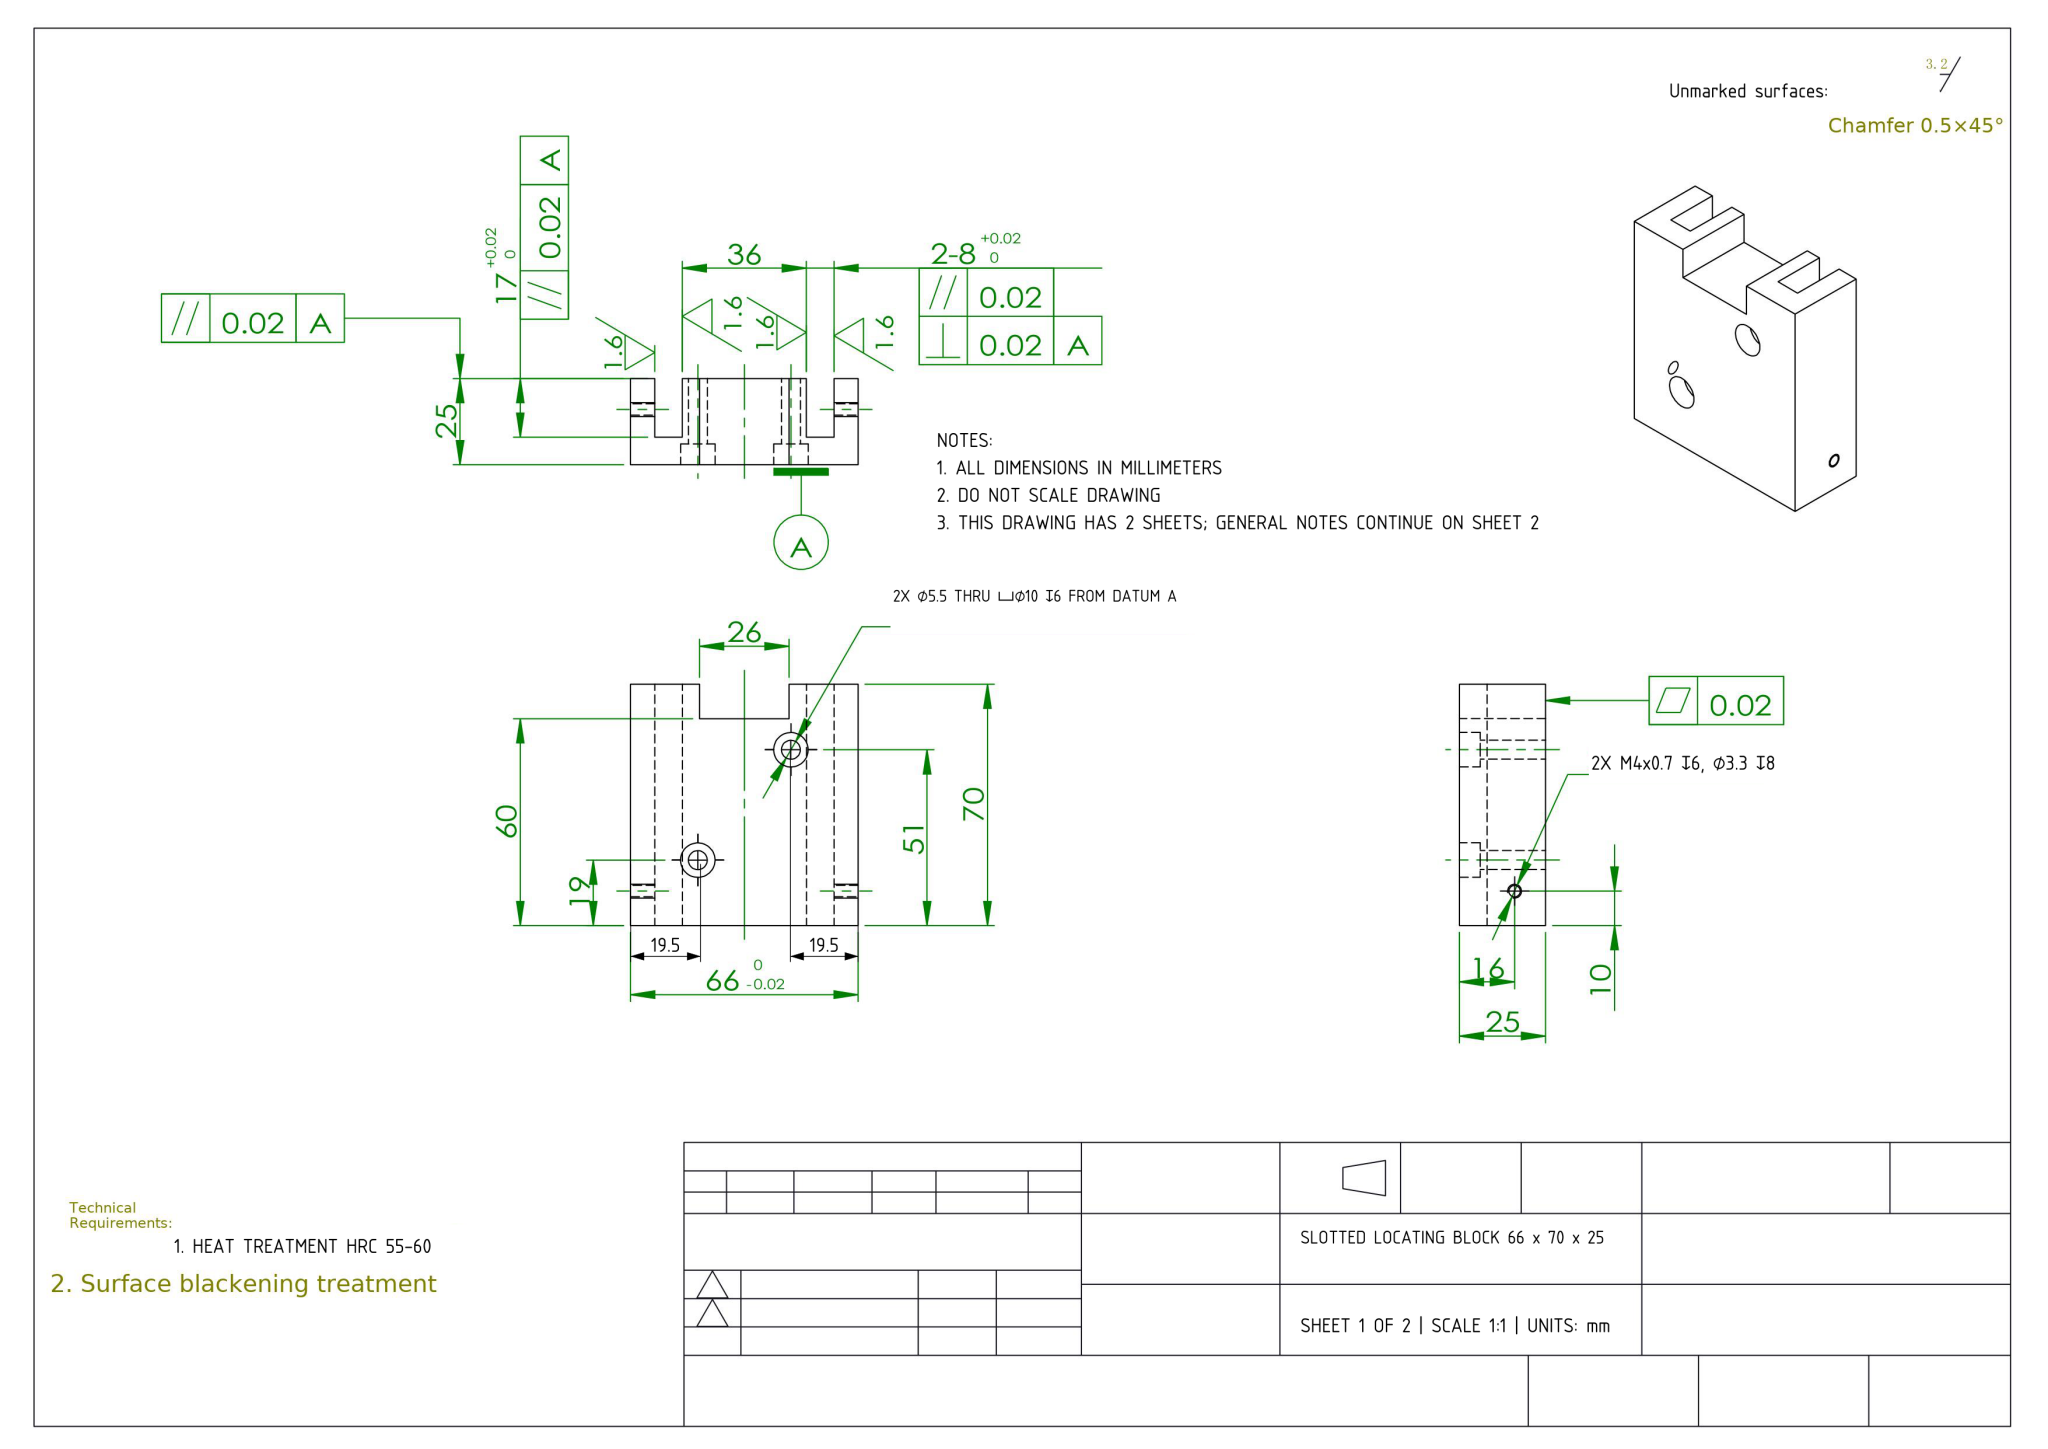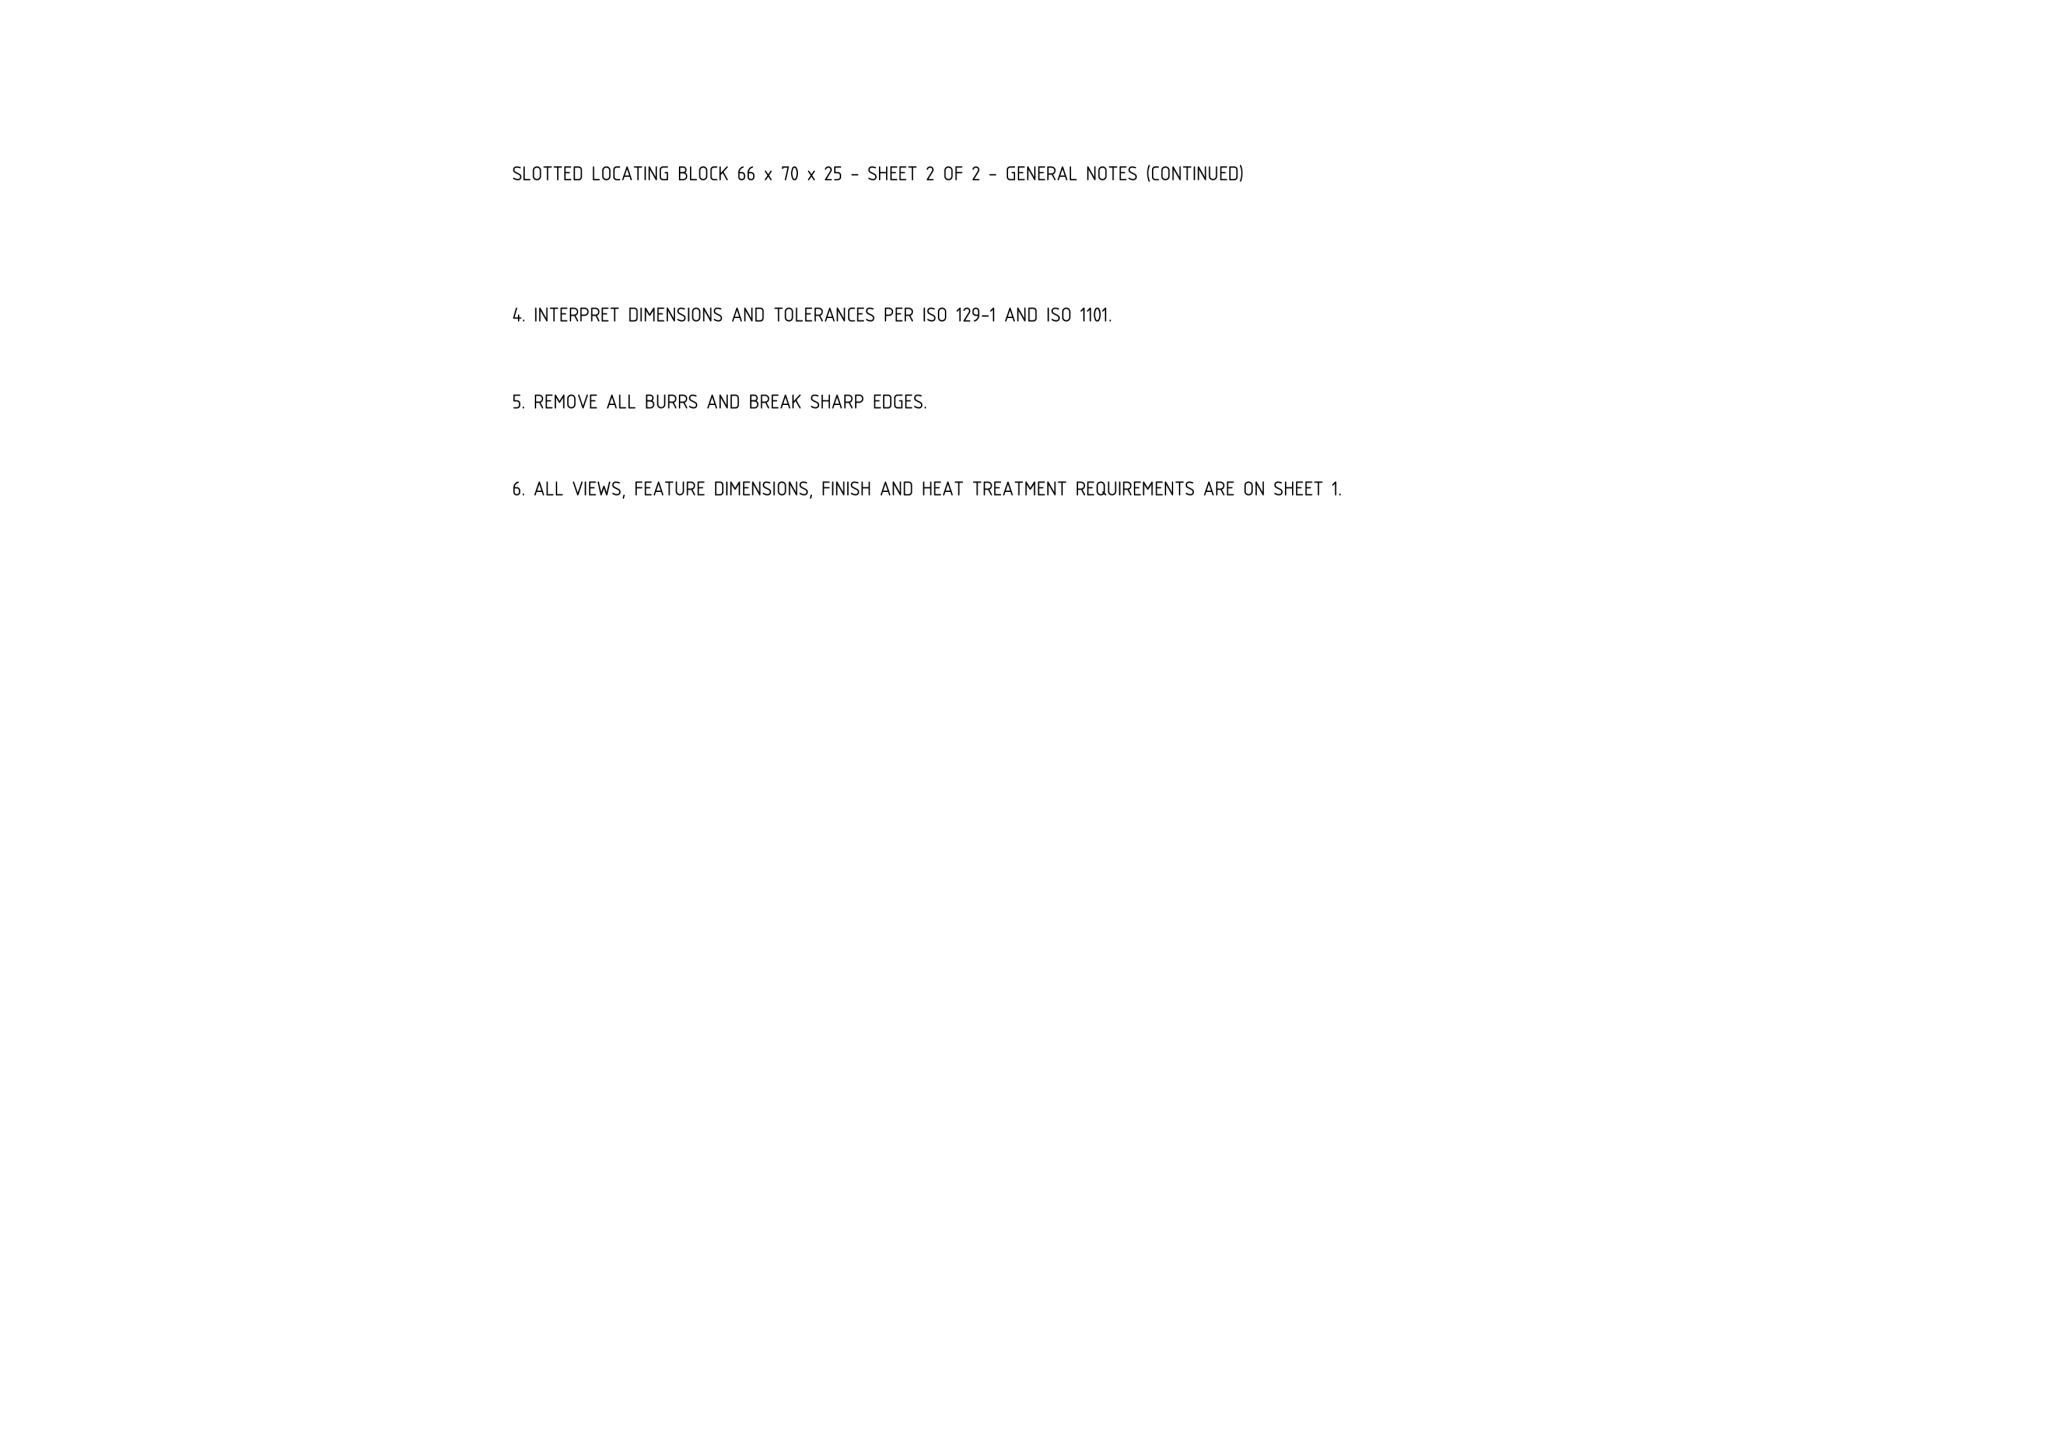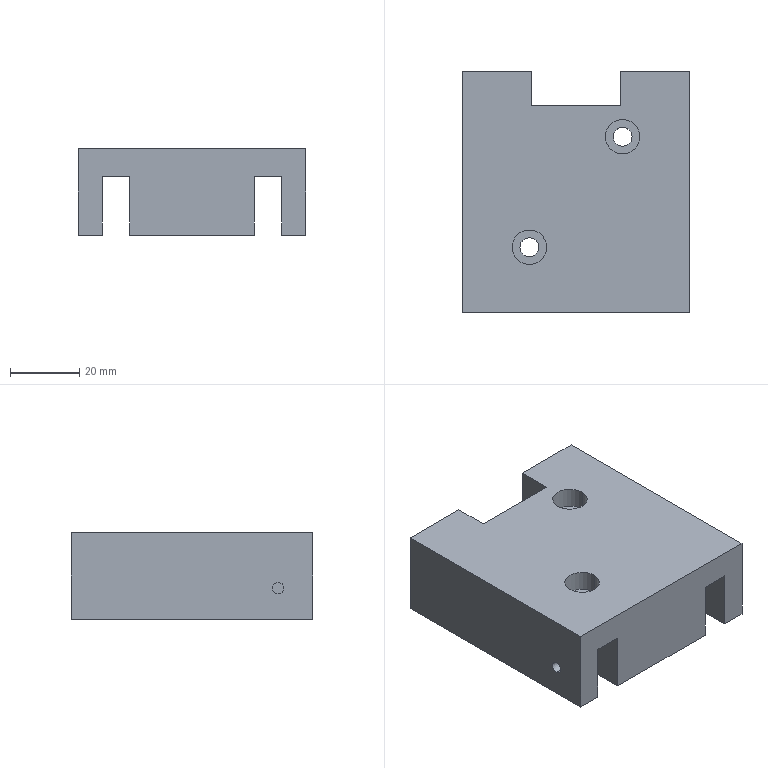Part | NX | mm | 1 solid | 32 faces | box 66 x 70 x 25 mm | volume 87995 mm3 | plane 20 | cylinder 12 | commonest cylinder face diameters 3.3 x4 5.5 x4 10 x4